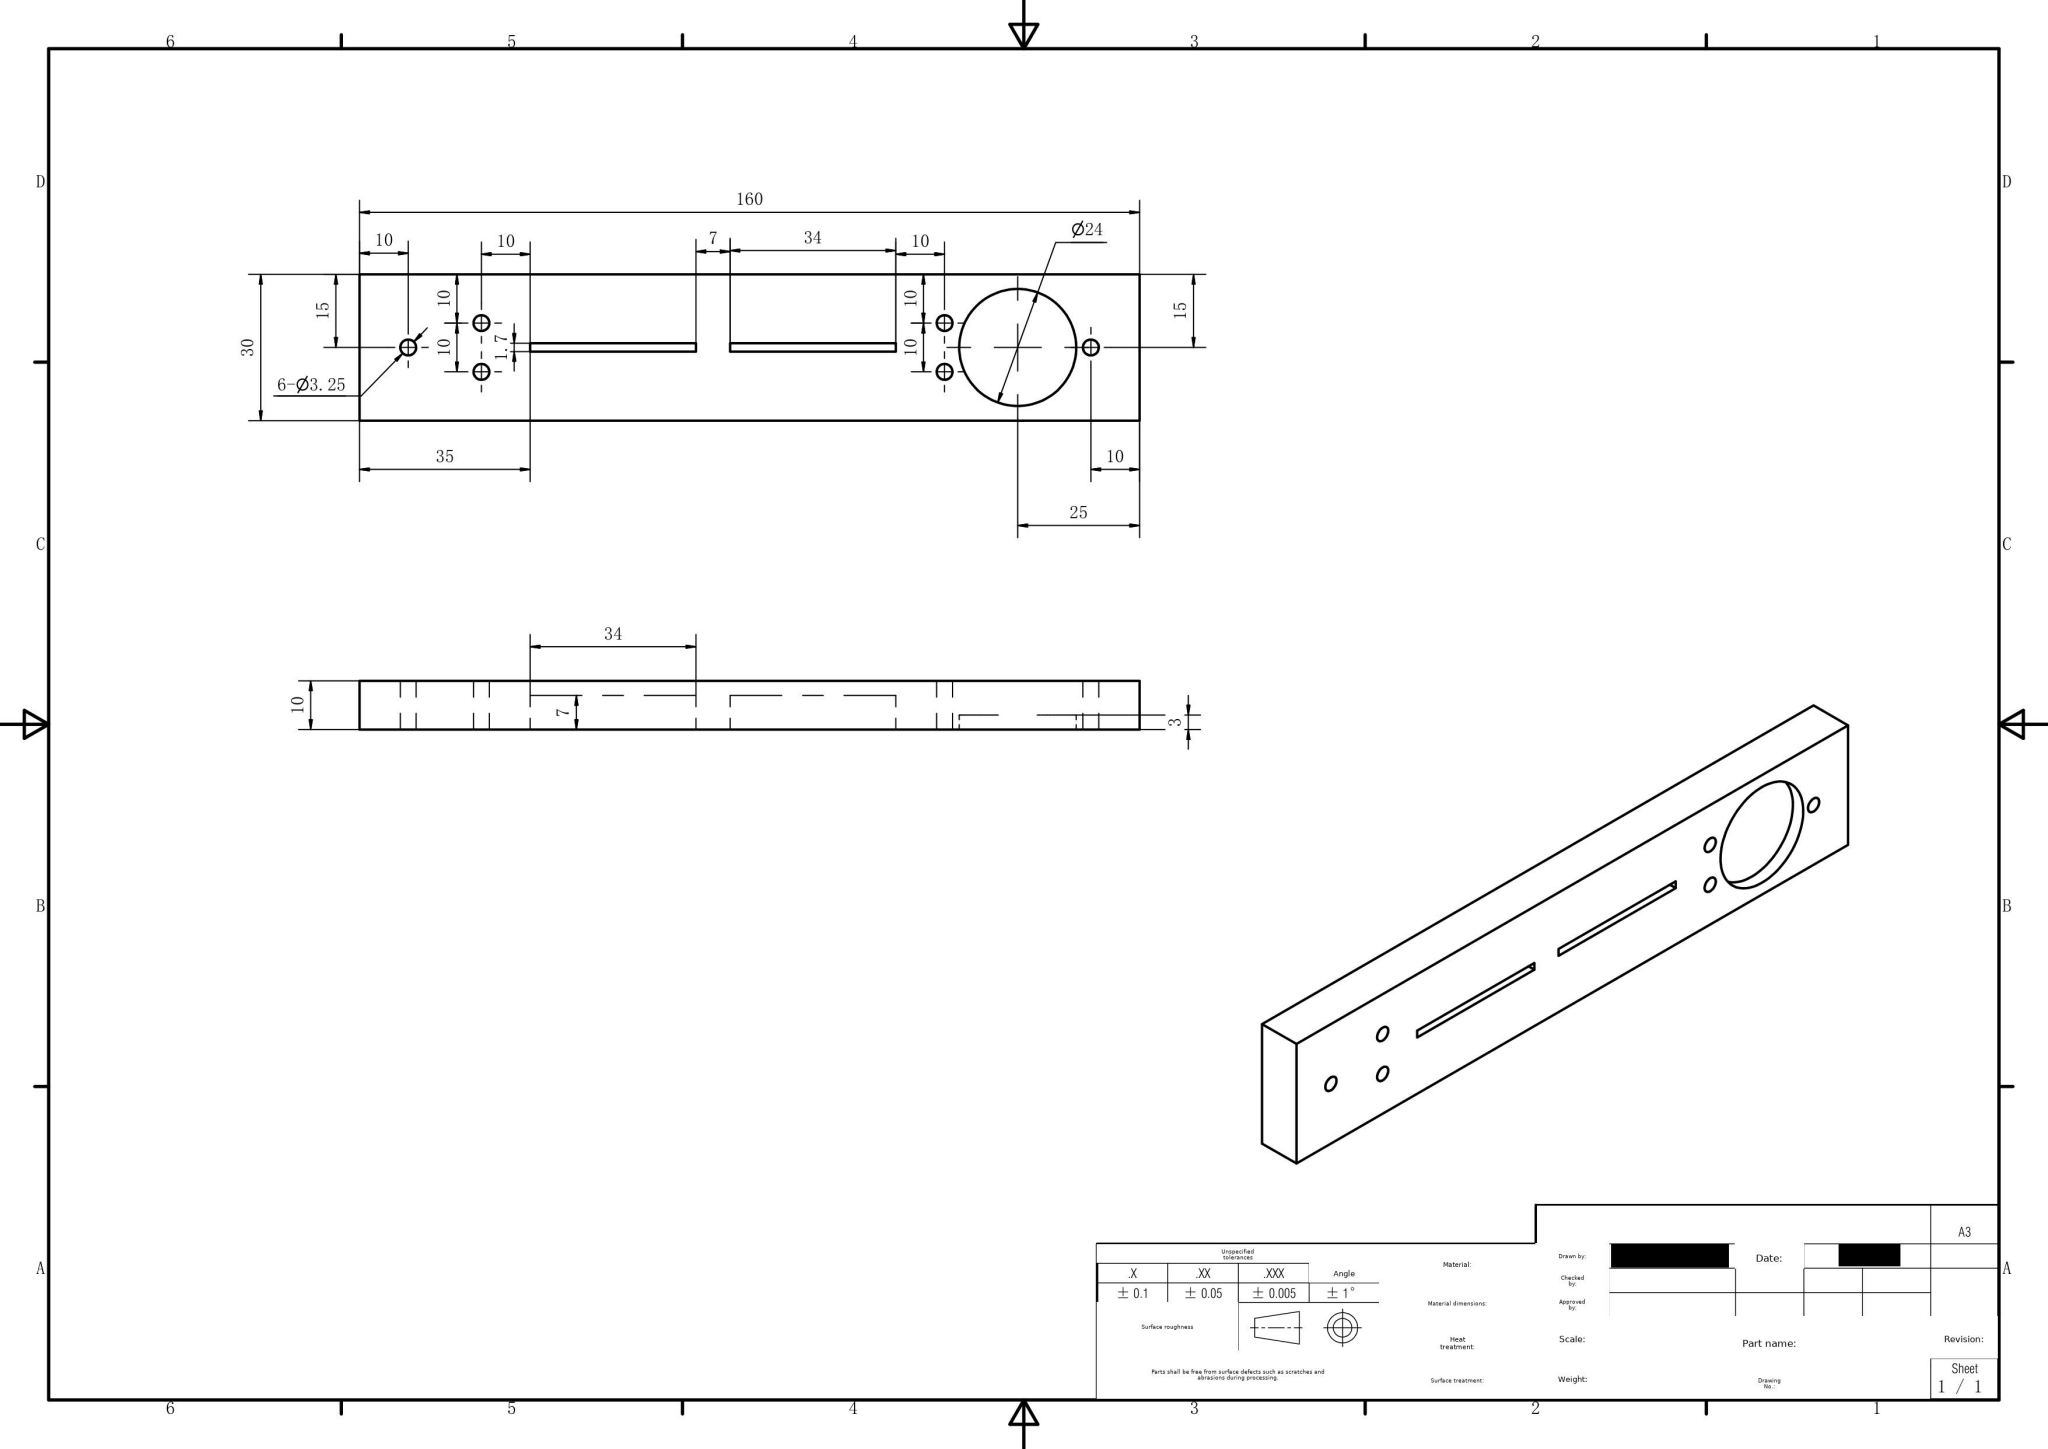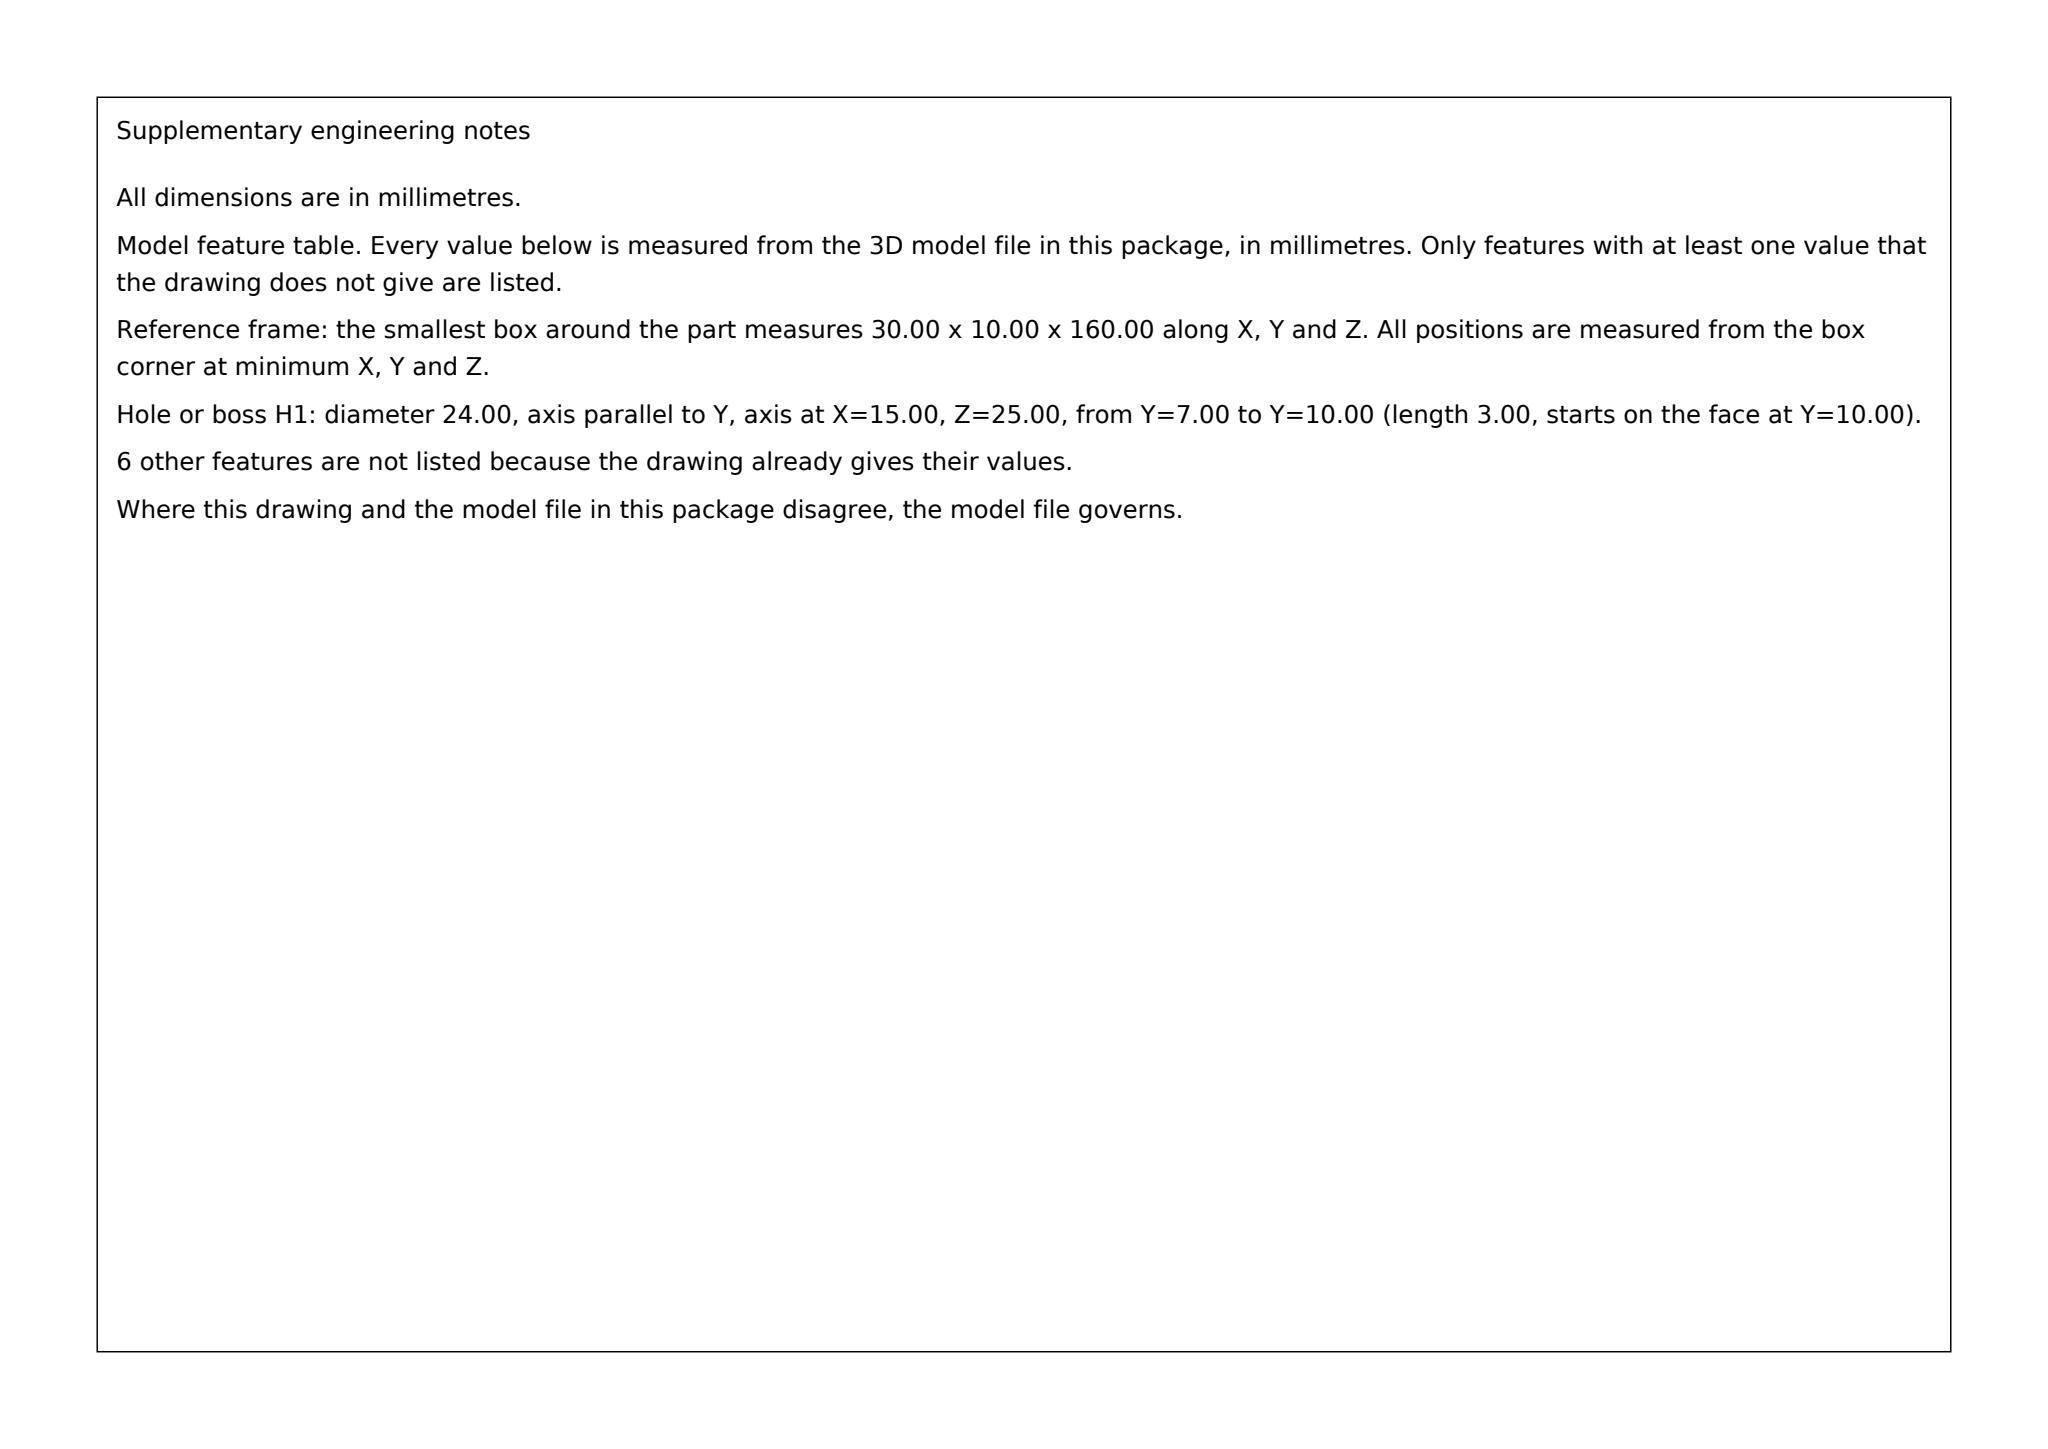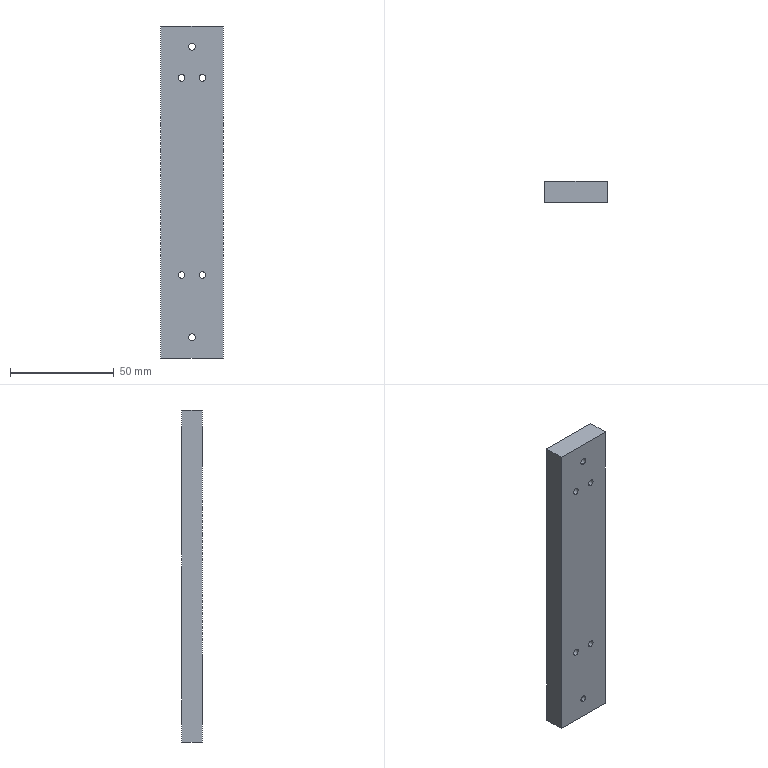Part | SolidWorks | mm | 1 solid | 31 faces | box 30 x 10 x 160 mm | volume 45336 mm3 | plane 17 | cylinder 14 | commonest cylinder face diameters 3.25 x12 24 x2